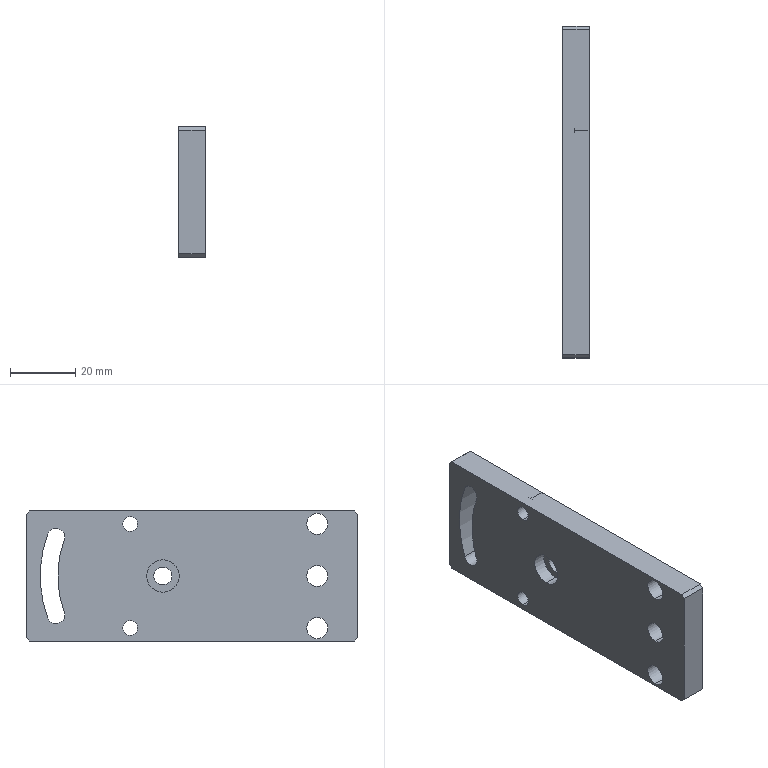Component | SolidWorks | MTCTV2104DJ006-000-0039Trimmer-1 | 1 solid | 36 faces | box 8 x 102 x 40 mm | volume 29621 mm3 | cylinder 23 | plane 13 | commonest cylinder face diameters 6.5 x6 7.9 x4 4.5 x4 5.4 x3 10 x2 5.5 x2 75.4 x1 64.6 x1
build123d program:
from build123d import *

# Parameters (mm, degrees)
SKETCH1_W                                           = 40
SKETCH1_H                                           = 52
BOSS_EXTRUDE1_DEPTH                                 = 8
HOLE_SIZE_TYPE_OF_HEXAGON_SOCKET_HEAD_C_D           = 5.5
HOLE_SIZE_TYPE_OF_HEXAGON_SOCKET_HEAD_C_CBORE_D     = 9.8
HOLE_SIZE_TYPE_OF_HEXAGON_SOCKET_HEAD_C_CBORE_DEPTH = 5.5
SKETCH14_W                                          = 8
SKETCH14_H                                          = 40
BOSS_EXTRUDE2_DEPTH                                 = 45
F_6_5_6_5_DIAMETER_HOLE1_D                          = 6.5
HOLE_SIZE_ACCORDING_TO_TYPE_3_OF_HEXA_D             = 4.5
HOLE_SIZE_ACCORDING_TO_TYPE_3_OF_HEXA_CBORE_D       = 7.9
HOLE_SIZE_ACCORDING_TO_TYPE_3_OF_HEXA_CBORE_DEPTH   = 4.6
SKETCH19_W                                          = 8
SKETCH19_H                                          = 40
BOSS_EXTRUDE3_DEPTH                                 = 10
CUT_EXTRUDE1_DEPTH                                  = 75.196
SKETCH20_W                                          = 8
SKETCH20_H                                          = 40
CUT_EXTRUDE2_DEPTH                                  = 5
SKETCH21_R                                          = 4.9
BOSS_EXTRUDE4_DEPTH                                 = 8
HOLE_SIZE_ACCORDING_TO_TYPE_4_OF_HEXA_D             = 5.5
HOLE_SIZE_ACCORDING_TO_TYPE_4_OF_HEXA_DEPTH         = 10.1
HOLE_SIZE_ACCORDING_TO_TYPE_4_OF_HEXA_CBORE_D       = 10
HOLE_SIZE_ACCORDING_TO_TYPE_4_OF_HEXA_CBORE_DEPTH   = 4
HOLE_SIZE_ACCORDING_TO_TYPE_4_OF_HEXA_TIP           = 1.652
CHAMFER1_SIZE                                       = 1
SKETCH24_W                                          = 40
SKETCH24_H                                          = 12.877
BOSS_EXTRUDE5_DEPTH                                 = 8
CUT_EXTRUDE3_DEPTH                                  = 75.196


with BuildPart() as part:
    # Sketch1 → Boss-Extrude1 (new body)
    with BuildSketch(Plane(origin=(0, 0, 0), x_dir=(0, 0, -1), z_dir=(1, 0, 0))):
        Rectangle(SKETCH1_W, SKETCH1_H)
    extrude(amount=BOSS_EXTRUDE1_DEPTH)

    # Hole Size _Type of Hexagon Socket Head C (through all)
    with Locations(Plane(origin=(8, 0, 0), x_dir=(0, 0, -1), z_dir=(1, 0, 0))):
        with Locations((0, 0)):
            CounterBoreHole(HOLE_SIZE_TYPE_OF_HEXAGON_SOCKET_HEAD_C_D / 2, HOLE_SIZE_TYPE_OF_HEXAGON_SOCKET_HEAD_C_CBORE_D / 2, HOLE_SIZE_TYPE_OF_HEXAGON_SOCKET_HEAD_C_CBORE_DEPTH)

    # Sketch14 → Boss-Extrude2 (add)
    with BuildSketch(Plane.XZ.offset(26)):
        with Locations((4, 0)):
            Rectangle(SKETCH14_W, SKETCH14_H)
    extrude(amount=BOSS_EXTRUDE2_DEPTH)

    # 6.5 _6.5_ Diameter Hole1 (through all)
    with Locations(Plane(origin=(8, 0, 0), x_dir=(0, 0, -1), z_dir=(1, 0, 0))):
        with Locations((16, -58.5), (0, -58.5), (-16, -58.5)):
            Hole(F_6_5_6_5_DIAMETER_HOLE1_D / 2)

    # Hole Size _ according to_ type 3 of Hexa (through all)
    with Locations(Plane.ZY):
        with Locations((-16, -1), (16, -1)):
            CounterBoreHole(HOLE_SIZE_ACCORDING_TO_TYPE_3_OF_HEXA_D / 2, HOLE_SIZE_ACCORDING_TO_TYPE_3_OF_HEXA_CBORE_D / 2, HOLE_SIZE_ACCORDING_TO_TYPE_3_OF_HEXA_CBORE_DEPTH)

    # Sketch19 → Boss-Extrude3 (add)
    with BuildSketch(Plane(origin=(0, 26, 0), x_dir=(1, 0, 0), z_dir=(0, 1, 0))):
        with Locations((4, 0)):
            Rectangle(SKETCH19_W, SKETCH19_H)
    extrude(amount=BOSS_EXTRUDE3_DEPTH)

    # Sketch9 → Cut-Extrude1 (cut, through all)
    with BuildSketch(Plane(origin=(8, 0, 0), x_dir=(0, 0, -1), z_dir=(1, 0, 0))):
        with BuildLine():
            ThreePointArc((13.85, 23.989), (0, 27.7), (-13.85, 23.989))
            ThreePointArc((-13.85, 23.989), (-14.838, 20.301), (-11.15, 19.312))
            ThreePointArc((-11.15, 19.312), (0, 22.3), (11.15, 19.312))
            ThreePointArc((11.15, 19.312), (14.838, 20.301), (13.85, 23.989))
        make_face()
    extrude(amount=-CUT_EXTRUDE1_DEPTH, mode=Mode.SUBTRACT)

    # Sketch20 → Cut-Extrude2 (cut)
    with BuildSketch(Plane(origin=(0, 36, 0), x_dir=(1, 0, 0), z_dir=(0, 1, 0))):
        with Locations((4, 0)):
            Rectangle(SKETCH20_W, SKETCH20_H)
    extrude(amount=-CUT_EXTRUDE2_DEPTH, mode=Mode.SUBTRACT)

    # Sketch21 → Boss-Extrude4 (add, through all)
    with BuildSketch(Plane(origin=(8, 0, 0), x_dir=(0, 0, -1), z_dir=(1, 0, 0))):
        Circle(SKETCH21_R)
    extrude(amount=-BOSS_EXTRUDE4_DEPTH)

    # Hole Size _ according to_ type 4 of Hexa
    with Locations(Plane(origin=(8, 0, 0), x_dir=(0, 0, -1), z_dir=(1, 0, 0))):
        with Locations((0, -11.041)):
            CounterBoreHole(HOLE_SIZE_ACCORDING_TO_TYPE_4_OF_HEXA_D / 2, HOLE_SIZE_ACCORDING_TO_TYPE_4_OF_HEXA_CBORE_D / 2, HOLE_SIZE_ACCORDING_TO_TYPE_4_OF_HEXA_CBORE_DEPTH, depth=HOLE_SIZE_ACCORDING_TO_TYPE_4_OF_HEXA_DEPTH)
            with Locations((0, 0, -(HOLE_SIZE_ACCORDING_TO_TYPE_4_OF_HEXA_DEPTH + HOLE_SIZE_ACCORDING_TO_TYPE_4_OF_HEXA_TIP / 2))):  # 118° drill point
                Cone(0, HOLE_SIZE_ACCORDING_TO_TYPE_4_OF_HEXA_D / 2, HOLE_SIZE_ACCORDING_TO_TYPE_4_OF_HEXA_TIP, mode=Mode.SUBTRACT)

    # Chamfer1
    chamfer1_edges = [part.edges().sort_by_distance(p)[0] for p in [
        (4, -71, 20),
        (4, -71, -20),
        (4, 31, 20),
        (4, 31, -20),
    ]]
    chamfer(chamfer1_edges, length=CHAMFER1_SIZE)

    # Sketch24 → Boss-Extrude5 (add, through all)
    with BuildSketch(Plane(origin=(8, 0, 0), x_dir=(0, 0, -1), z_dir=(1, 0, 0))):
        with Locations((0, 23.562)):
            Rectangle(SKETCH24_W, SKETCH24_H)
    extrude(amount=-BOSS_EXTRUDE5_DEPTH)

    # Sketch25 → Cut-Extrude3 (cut, through all)
    with BuildSketch(Plane(origin=(8, 0, 0), x_dir=(0, 0, -1), z_dir=(1, 0, 0))):
        with BuildLine():
            ThreePointArc((12.894, 24.385), (0, 26.659), (-12.894, 24.385))
            ThreePointArc((-12.894, 24.385), (-14.508, 20.925), (-11.047, 19.311))
            ThreePointArc((-11.047, 19.311), (0, 21.259), (11.047, 19.311))
            ThreePointArc((11.047, 19.311), (14.508, 20.925), (12.894, 24.385))
        make_face()
    extrude(amount=-CUT_EXTRUDE3_DEPTH, mode=Mode.SUBTRACT)


solid = part.part

# Placed as in the assembly
solid = solid.moved(Location((39.798, -29.678, 265.447), (-180, 0, 180)))